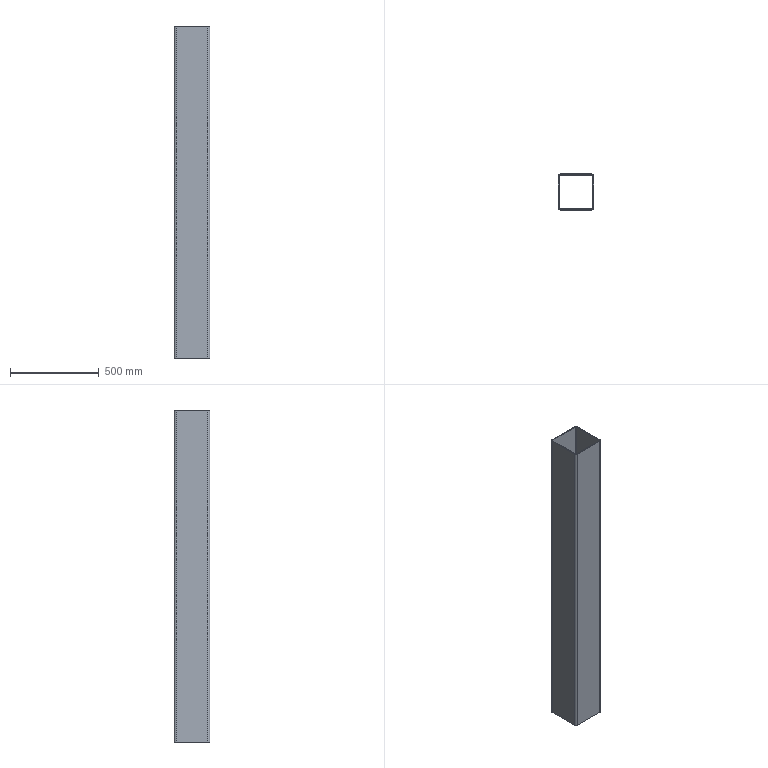Component | SolidWorks | 200 x 200 x 5-1 | 1 solid | 18 faces | box 200 x 200 x 1874 mm | volume 7187951 mm3 | plane 10 | cylinder 8 | commonest cylinder face diameters 20 x4 10 x4 | material Plain Carbon Steel
build123d program:
from build123d import *

# Parameters (mm, degrees)
BOSS_EXTRUDE1_DEPTH = 1874


with BuildPart() as part:
    # Sketch1 → Boss-Extrude1 (new body)
    with BuildSketch(Plane.XY):
        with BuildLine():
            Line((-90, -100), (90, -100))
            ThreePointArc((90, -100), (97.071, -97.071), (100, -90))
            Line((100, -90), (100, 90))
            ThreePointArc((100, 90), (97.071, 97.071), (90, 100))
            Line((90, 100), (-90, 100))
            ThreePointArc((-90, 100), (-97.071, 97.071), (-100, 90))
            Line((-100, 90), (-100, -90))
            ThreePointArc((-100, -90), (-97.071, -97.071), (-90, -100))
        make_face()
        with BuildLine():
            Line((-90, -95), (90, -95))
            ThreePointArc((90, -95), (93.536, -93.536), (95, -90))
            Line((95, -90), (95, 90))
            ThreePointArc((95, 90), (93.536, 93.536), (90, 95))
            Line((90, 95), (-90, 95))
            ThreePointArc((-90, 95), (-93.536, 93.536), (-95, 90))
            Line((-95, 90), (-95, -90))
            ThreePointArc((-95, -90), (-93.536, -93.536), (-90, -95))
        make_face(mode=Mode.SUBTRACT)
    extrude(amount=BOSS_EXTRUDE1_DEPTH)


solid = part.part

# Placed as in the assembly
solid = solid.moved(Location((585.937, 2371.697, 1863.287), (0, 0, 0)))
STEP:
#1=CARTESIAN_POINT('',(19.131,89.831,147.137));
#2=VERTEX_POINT('',#1);
#3=CARTESIAN_POINT('',(19.525,89.437,147.137));
#4=VERTEX_POINT('',#3);
#5=CARTESIAN_POINT('',(19.525,89.831,147.137));
#6=DIRECTION('',(0.,0.,1.));
#7=DIRECTION('',(1.,0.,0.));
#8=AXIS2_PLACEMENT_3D('',#5,#6,#7);
#9=CIRCLE('',#8,0.3937);
#10=EDGE_CURVE('',#2,#4,#9,.T.);
#11=ORIENTED_EDGE('',*,*,#10,.T.);
#12=CARTESIAN_POINT('',(26.612,89.437,147.137));
#13=VERTEX_POINT('',#12);
#14=CARTESIAN_POINT('',(19.525,89.437,147.137));
#15=DIRECTION('',(1.,0.,0.));
#16=VECTOR('',#15,39.37);
#17=LINE('',#14,#16);
#18=EDGE_CURVE('',#4,#13,#17,.T.);
#19=ORIENTED_EDGE('',*,*,#18,.T.);
#20=CARTESIAN_POINT('',(27.005,89.831,147.137));
#21=VERTEX_POINT('',#20);
#22=CARTESIAN_POINT('',(26.612,89.831,147.137));
#23=DIRECTION('',(0.,0.,1.));
#24=DIRECTION('',(1.,0.,0.));
#25=AXIS2_PLACEMENT_3D('',#22,#23,#24);
#26=CIRCLE('',#25,0.3937);
#27=EDGE_CURVE('',#13,#21,#26,.T.);
#28=ORIENTED_EDGE('',*,*,#27,.T.);
#29=CARTESIAN_POINT('',(27.005,96.917,147.137));
#30=VERTEX_POINT('',#29);
#31=CARTESIAN_POINT('',(27.005,96.917,147.137));
#32=DIRECTION('',(0.,-1.,0.));
#33=VECTOR('',#32,39.37);
#34=LINE('',#31,#33);
#35=EDGE_CURVE('',#30,#21,#34,.T.);
#36=ORIENTED_EDGE('',*,*,#35,.F.);
#37=CARTESIAN_POINT('',(26.612,97.311,147.137));
#38=VERTEX_POINT('',#37);
#39=CARTESIAN_POINT('',(26.612,96.917,147.137));
#40=DIRECTION('',(0.,0.,1.));
#41=DIRECTION('',(1.,0.,0.));
#42=AXIS2_PLACEMENT_3D('',#39,#40,#41);
#43=CIRCLE('',#42,0.3937);
#44=EDGE_CURVE('',#30,#38,#43,.T.);
#45=ORIENTED_EDGE('',*,*,#44,.T.);
#46=CARTESIAN_POINT('',(19.525,97.311,147.137));
#47=VERTEX_POINT('',#46);
#48=CARTESIAN_POINT('',(26.612,97.311,147.137));
#49=DIRECTION('',(-1.,0.,0.));
#50=VECTOR('',#49,39.37);
#51=LINE('',#48,#50);
#52=EDGE_CURVE('',#38,#47,#51,.T.);
#53=ORIENTED_EDGE('',*,*,#52,.T.);
#54=CARTESIAN_POINT('',(19.131,96.917,147.137));
#55=VERTEX_POINT('',#54);
#56=CARTESIAN_POINT('',(19.525,96.917,147.137));
#57=DIRECTION('',(0.,0.,1.));
#58=DIRECTION('',(1.,0.,0.));
#59=AXIS2_PLACEMENT_3D('',#56,#57,#58);
#60=CIRCLE('',#59,0.3937);
#61=EDGE_CURVE('',#47,#55,#60,.T.);
#62=ORIENTED_EDGE('',*,*,#61,.T.);
#63=CARTESIAN_POINT('',(19.131,89.831,147.137));
#64=DIRECTION('',(0.,1.,0.));
#65=VECTOR('',#64,39.37);
#66=LINE('',#63,#65);
#67=EDGE_CURVE('',#2,#55,#66,.T.);
#68=ORIENTED_EDGE('',*,*,#67,.F.);
#69=EDGE_LOOP('',(#11,#19,#28,#36,#45,#53,#62,#68));
#70=FACE_OUTER_BOUND('',#69,.T.);
#71=CARTESIAN_POINT('',(19.525,89.634,147.137));
#72=VERTEX_POINT('',#71);
#73=CARTESIAN_POINT('',(26.612,89.634,147.137));
#74=VERTEX_POINT('',#73);
#75=CARTESIAN_POINT('',(19.525,89.634,147.137));
#76=DIRECTION('',(1.,0.,0.));
#77=VECTOR('',#76,39.37);
#78=LINE('',#75,#77);
#79=EDGE_CURVE('',#72,#74,#78,.T.);
#80=ORIENTED_EDGE('',*,*,#79,.F.);
#81=CARTESIAN_POINT('',(19.328,89.831,147.137));
#82=VERTEX_POINT('',#81);
#83=CARTESIAN_POINT('',(19.525,89.831,147.137));
#84=DIRECTION('',(0.,0.,1.));
#85=DIRECTION('',(1.,0.,0.));
#86=AXIS2_PLACEMENT_3D('',#83,#84,#85);
#87=CIRCLE('',#86,0.1969);
#88=EDGE_CURVE('',#82,#72,#87,.T.);
#89=ORIENTED_EDGE('',*,*,#88,.F.);
#90=CARTESIAN_POINT('',(19.328,96.917,147.137));
#91=VERTEX_POINT('',#90);
#92=CARTESIAN_POINT('',(19.328,89.831,147.137));
#93=DIRECTION('',(0.,1.,0.));
#94=VECTOR('',#93,39.37);
#95=LINE('',#92,#94);
#96=EDGE_CURVE('',#82,#91,#95,.T.);
#97=ORIENTED_EDGE('',*,*,#96,.T.);
#98=CARTESIAN_POINT('',(19.525,97.114,147.137));
#99=VERTEX_POINT('',#98);
#100=CARTESIAN_POINT('',(19.525,96.917,147.137));
#101=DIRECTION('',(0.,0.,1.));
#102=DIRECTION('',(1.,0.,0.));
#103=AXIS2_PLACEMENT_3D('',#100,#101,#102);
#104=CIRCLE('',#103,0.1969);
#105=EDGE_CURVE('',#99,#91,#104,.T.);
#106=ORIENTED_EDGE('',*,*,#105,.F.);
#107=CARTESIAN_POINT('',(26.612,97.114,147.137));
#108=VERTEX_POINT('',#107);
#109=CARTESIAN_POINT('',(26.612,97.114,147.137));
#110=DIRECTION('',(-1.,0.,0.));
#111=VECTOR('',#110,39.37);
#112=LINE('',#109,#111);
#113=EDGE_CURVE('',#108,#99,#112,.T.);
#114=ORIENTED_EDGE('',*,*,#113,.F.);
#115=CARTESIAN_POINT('',(26.809,96.917,147.137));
#116=VERTEX_POINT('',#115);
#117=CARTESIAN_POINT('',(26.612,96.917,147.137));
#118=DIRECTION('',(0.,0.,1.));
#119=DIRECTION('',(1.,0.,0.));
#120=AXIS2_PLACEMENT_3D('',#117,#118,#119);
#121=CIRCLE('',#120,0.1969);
#122=EDGE_CURVE('',#116,#108,#121,.T.);
#123=ORIENTED_EDGE('',*,*,#122,.F.);
#124=CARTESIAN_POINT('',(26.809,89.831,147.137));
#125=VERTEX_POINT('',#124);
#126=CARTESIAN_POINT('',(26.809,96.917,147.137));
#127=DIRECTION('',(0.,-1.,0.));
#128=VECTOR('',#127,39.37);
#129=LINE('',#126,#128);
#130=EDGE_CURVE('',#116,#125,#129,.T.);
#131=ORIENTED_EDGE('',*,*,#130,.T.);
#132=CARTESIAN_POINT('',(26.612,89.831,147.137));
#133=DIRECTION('',(0.,0.,1.));
#134=DIRECTION('',(1.,0.,0.));
#135=AXIS2_PLACEMENT_3D('',#132,#133,#134);
#136=CIRCLE('',#135,0.1969);
#137=EDGE_CURVE('',#74,#125,#136,.T.);
#138=ORIENTED_EDGE('',*,*,#137,.F.);
#139=EDGE_LOOP('',(#80,#89,#97,#106,#114,#123,#131,#138));
#140=FACE_BOUND('',#139,.T.);
#141=CARTESIAN_POINT('',(19.525,89.831,147.137));
#142=DIRECTION('',(0.,0.,1.));
#143=DIRECTION('',(1.,0.,0.));
#144=AXIS2_PLACEMENT_3D('',#141,#142,#143);
#145=PLANE('',#144);
#146=ADVANCED_FACE('',(#70,#140),#145,.T.);
#147=CARTESIAN_POINT('',(19.131,89.831,73.358));
#148=VERTEX_POINT('',#147);
#149=CARTESIAN_POINT('',(19.525,89.437,73.358));
#150=VERTEX_POINT('',#149);
#151=CARTESIAN_POINT('',(19.525,89.831,73.358));
#152=DIRECTION('',(0.,0.,1.));
#153=DIRECTION('',(1.,0.,0.));
#154=AXIS2_PLACEMENT_3D('',#151,#152,#153);
#155=CIRCLE('',#154,0.3937);
#156=EDGE_CURVE('',#148,#150,#155,.T.);
#157=ORIENTED_EDGE('',*,*,#156,.F.);
#158=CARTESIAN_POINT('',(19.131,96.917,73.358));
#159=VERTEX_POINT('',#158);
#160=CARTESIAN_POINT('',(19.131,89.831,73.358));
#161=DIRECTION('',(0.,1.,0.));
#162=VECTOR('',#161,39.37);
#163=LINE('',#160,#162);
#164=EDGE_CURVE('',#148,#159,#163,.T.);
#165=ORIENTED_EDGE('',*,*,#164,.T.);
#166=CARTESIAN_POINT('',(19.525,97.311,73.358));
#167=VERTEX_POINT('',#166);
#168=CARTESIAN_POINT('',(19.525,96.917,73.358));
#169=DIRECTION('',(0.,0.,1.));
#170=DIRECTION('',(1.,0.,0.));
#171=AXIS2_PLACEMENT_3D('',#168,#169,#170);
#172=CIRCLE('',#171,0.3937);
#173=EDGE_CURVE('',#167,#159,#172,.T.);
#174=ORIENTED_EDGE('',*,*,#173,.F.);
#175=CARTESIAN_POINT('',(26.612,97.311,73.358));
#176=VERTEX_POINT('',#175);
#177=CARTESIAN_POINT('',(26.612,97.311,73.358));
#178=DIRECTION('',(-1.,0.,0.));
#179=VECTOR('',#178,39.37);
#180=LINE('',#177,#179);
#181=EDGE_CURVE('',#176,#167,#180,.T.);
#182=ORIENTED_EDGE('',*,*,#181,.F.);
#183=CARTESIAN_POINT('',(27.005,96.917,73.358));
#184=VERTEX_POINT('',#183);
#185=CARTESIAN_POINT('',(26.612,96.917,73.358));
#186=DIRECTION('',(0.,0.,1.));
#187=DIRECTION('',(1.,0.,0.));
#188=AXIS2_PLACEMENT_3D('',#185,#186,#187);
#189=CIRCLE('',#188,0.3937);
#190=EDGE_CURVE('',#184,#176,#189,.T.);
#191=ORIENTED_EDGE('',*,*,#190,.F.);
#192=CARTESIAN_POINT('',(27.005,89.831,73.358));
#193=VERTEX_POINT('',#192);
#194=CARTESIAN_POINT('',(27.005,96.917,73.358));
#195=DIRECTION('',(0.,-1.,0.));
#196=VECTOR('',#195,39.37);
#197=LINE('',#194,#196);
#198=EDGE_CURVE('',#184,#193,#197,.T.);
#199=ORIENTED_EDGE('',*,*,#198,.T.);
#200=CARTESIAN_POINT('',(26.612,89.437,73.358));
#201=VERTEX_POINT('',#200);
#202=CARTESIAN_POINT('',(26.612,89.831,73.358));
#203=DIRECTION('',(0.,0.,1.));
#204=DIRECTION('',(1.,0.,0.));
#205=AXIS2_PLACEMENT_3D('',#202,#203,#204);
#206=CIRCLE('',#205,0.3937);
#207=EDGE_CURVE('',#201,#193,#206,.T.);
#208=ORIENTED_EDGE('',*,*,#207,.F.);
#209=CARTESIAN_POINT('',(19.525,89.437,73.358));
#210=DIRECTION('',(1.,0.,0.));
#211=VECTOR('',#210,39.37);
#212=LINE('',#209,#211);
#213=EDGE_CURVE('',#150,#201,#212,.T.);
#214=ORIENTED_EDGE('',*,*,#213,.F.);
#215=EDGE_LOOP('',(#157,#165,#174,#182,#191,#199,#208,#214));
#216=FACE_OUTER_BOUND('',#215,.T.);
#217=CARTESIAN_POINT('',(19.328,89.831,73.358));
#218=VERTEX_POINT('',#217);
#219=CARTESIAN_POINT('',(19.525,89.634,73.358));
#220=VERTEX_POINT('',#219);
#221=CARTESIAN_POINT('',(19.525,89.831,73.358));
#222=DIRECTION('',(0.,0.,1.));
#223=DIRECTION('',(1.,0.,0.));
#224=AXIS2_PLACEMENT_3D('',#221,#222,#223);
#225=CIRCLE('',#224,0.1969);
#226=EDGE_CURVE('',#218,#220,#225,.T.);
#227=ORIENTED_EDGE('',*,*,#226,.T.);
#228=CARTESIAN_POINT('',(26.612,89.634,73.358));
#229=VERTEX_POINT('',#228);
#230=CARTESIAN_POINT('',(19.525,89.634,73.358));
#231=DIRECTION('',(1.,0.,0.));
#232=VECTOR('',#231,39.37);
#233=LINE('',#230,#232);
#234=EDGE_CURVE('',#220,#229,#233,.T.);
#235=ORIENTED_EDGE('',*,*,#234,.T.);
#236=CARTESIAN_POINT('',(26.809,89.831,73.358));
#237=VERTEX_POINT('',#236);
#238=CARTESIAN_POINT('',(26.612,89.831,73.358));
#239=DIRECTION('',(0.,0.,1.));
#240=DIRECTION('',(1.,0.,0.));
#241=AXIS2_PLACEMENT_3D('',#238,#239,#240);
#242=CIRCLE('',#241,0.1969);
#243=EDGE_CURVE('',#229,#237,#242,.T.);
#244=ORIENTED_EDGE('',*,*,#243,.T.);
#245=CARTESIAN_POINT('',(26.809,96.917,73.358));
#246=VERTEX_POINT('',#245);
#247=CARTESIAN_POINT('',(26.809,96.917,73.358));
#248=DIRECTION('',(0.,-1.,0.));
#249=VECTOR('',#248,39.37);
#250=LINE('',#247,#249);
#251=EDGE_CURVE('',#246,#237,#250,.T.);
#252=ORIENTED_EDGE('',*,*,#251,.F.);
#253=CARTESIAN_POINT('',(26.612,97.114,73.358));
#254=VERTEX_POINT('',#253);
#255=CARTESIAN_POINT('',(26.612,96.917,73.358));
#256=DIRECTION('',(0.,0.,1.));
#257=DIRECTION('',(1.,0.,0.));
#258=AXIS2_PLACEMENT_3D('',#255,#256,#257);
#259=CIRCLE('',#258,0.1969);
#260=EDGE_CURVE('',#246,#254,#259,.T.);
#261=ORIENTED_EDGE('',*,*,#260,.T.);
#262=CARTESIAN_POINT('',(19.525,97.114,73.358));
#263=VERTEX_POINT('',#262);
#264=CARTESIAN_POINT('',(26.612,97.114,73.358));
#265=DIRECTION('',(-1.,0.,0.));
#266=VECTOR('',#265,39.37);
#267=LINE('',#264,#266);
#268=EDGE_CURVE('',#254,#263,#267,.T.);
#269=ORIENTED_EDGE('',*,*,#268,.T.);
#270=CARTESIAN_POINT('',(19.328,96.917,73.358));
#271=VERTEX_POINT('',#270);
#272=CARTESIAN_POINT('',(19.525,96.917,73.358));
#273=DIRECTION('',(0.,0.,1.));
#274=DIRECTION('',(1.,0.,0.));
#275=AXIS2_PLACEMENT_3D('',#272,#273,#274);
#276=CIRCLE('',#275,0.1969);
#277=EDGE_CURVE('',#263,#271,#276,.T.);
#278=ORIENTED_EDGE('',*,*,#277,.T.);
#279=CARTESIAN_POINT('',(19.328,89.831,73.358));
#280=DIRECTION('',(0.,1.,0.));
#281=VECTOR('',#280,39.37);
#282=LINE('',#279,#281);
#283=EDGE_CURVE('',#218,#271,#282,.T.);
#284=ORIENTED_EDGE('',*,*,#283,.F.);
#285=EDGE_LOOP('',(#227,#235,#244,#252,#261,#269,#278,#284));
#286=FACE_BOUND('',#285,.T.);
#287=CARTESIAN_POINT('',(19.525,89.831,73.358));
#288=DIRECTION('',(0.,0.,1.));
#289=DIRECTION('',(1.,0.,0.));
#290=AXIS2_PLACEMENT_3D('',#287,#288,#289);
#291=PLANE('',#290);
#292=ADVANCED_FACE('',(#216,#286),#291,.F.);
#293=ORIENTED_EDGE('',*,*,#156,.T.);
#294=CARTESIAN_POINT('',(19.525,89.437,147.137));
#295=DIRECTION('',(0.,0.,-1.));
#296=VECTOR('',#295,39.37);
#297=LINE('',#294,#296);
#298=EDGE_CURVE('',#4,#150,#297,.T.);
#299=ORIENTED_EDGE('',*,*,#298,.F.);
#300=ORIENTED_EDGE('',*,*,#10,.F.);
#301=CARTESIAN_POINT('',(19.131,89.831,147.137));
#302=DIRECTION('',(0.,0.,-1.));
#303=VECTOR('',#302,39.37);
#304=LINE('',#301,#303);
#305=EDGE_CURVE('',#2,#148,#304,.T.);
#306=ORIENTED_EDGE('',*,*,#305,.T.);
#307=EDGE_LOOP('',(#293,#299,#300,#306));
#308=FACE_OUTER_BOUND('',#307,.T.);
#309=CARTESIAN_POINT('',(19.525,89.831,147.137));
#310=DIRECTION('',(0.,0.,-1.));
#311=DIRECTION('',(-1.,0.,0.));
#312=AXIS2_PLACEMENT_3D('',#309,#310,#311);
#313=CYLINDRICAL_SURFACE('',#312,0.3937);
#314=ADVANCED_FACE('',(#308),#313,.T.);
#315=ORIENTED_EDGE('',*,*,#213,.T.);
#316=CARTESIAN_POINT('',(26.612,89.437,147.137));
#317=DIRECTION('',(0.,0.,-1.));
#318=VECTOR('',#317,39.37);
#319=LINE('',#316,#318);
#320=EDGE_CURVE('',#13,#201,#319,.T.);
#321=ORIENTED_EDGE('',*,*,#320,.F.);
#322=ORIENTED_EDGE('',*,*,#18,.F.);
#323=ORIENTED_EDGE('',*,*,#298,.T.);
#324=EDGE_LOOP('',(#315,#321,#322,#323));
#325=FACE_OUTER_BOUND('',#324,.T.);
#326=CARTESIAN_POINT('',(19.525,89.437,147.137));
#327=DIRECTION('',(0.,1.,0.));
#328=DIRECTION('',(0.,0.,1.));
#329=AXIS2_PLACEMENT_3D('',#326,#327,#328);
#330=PLANE('',#329);
#331=ADVANCED_FACE('',(#325),#330,.F.);
#332=ORIENTED_EDGE('',*,*,#207,.T.);
#333=CARTESIAN_POINT('',(27.005,89.831,147.137));
#334=DIRECTION('',(0.,0.,-1.));
#335=VECTOR('',#334,39.37);
#336=LINE('',#333,#335);
#337=EDGE_CURVE('',#21,#193,#336,.T.);
#338=ORIENTED_EDGE('',*,*,#337,.F.);
#339=ORIENTED_EDGE('',*,*,#27,.F.);
#340=ORIENTED_EDGE('',*,*,#320,.T.);
#341=EDGE_LOOP('',(#332,#338,#339,#340));
#342=FACE_OUTER_BOUND('',#341,.T.);
#343=CARTESIAN_POINT('',(26.612,89.831,147.137));
#344=DIRECTION('',(0.,0.,-1.));
#345=DIRECTION('',(-1.,0.,0.));
#346=AXIS2_PLACEMENT_3D('',#343,#344,#345);
#347=CYLINDRICAL_SURFACE('',#346,0.3937);
#348=ADVANCED_FACE('',(#342),#347,.T.);
#349=ORIENTED_EDGE('',*,*,#198,.F.);
#350=CARTESIAN_POINT('',(27.005,96.917,147.137));
#351=DIRECTION('',(0.,0.,-1.));
#352=VECTOR('',#351,39.37);
#353=LINE('',#350,#352);
#354=EDGE_CURVE('',#30,#184,#353,.T.);
#355=ORIENTED_EDGE('',*,*,#354,.F.);
#356=ORIENTED_EDGE('',*,*,#35,.T.);
#357=ORIENTED_EDGE('',*,*,#337,.T.);
#358=EDGE_LOOP('',(#349,#355,#356,#357));
#359=FACE_OUTER_BOUND('',#358,.T.);
#360=CARTESIAN_POINT('',(27.005,96.917,147.137));
#361=DIRECTION('',(1.,0.,0.));
#362=DIRECTION('',(0.,0.,-1.));
#363=AXIS2_PLACEMENT_3D('',#360,#361,#362);
#364=PLANE('',#363);
#365=ADVANCED_FACE('',(#359),#364,.T.);
#366=ORIENTED_EDGE('',*,*,#190,.T.);
#367=CARTESIAN_POINT('',(26.612,97.311,147.137));
#368=DIRECTION('',(0.,0.,-1.));
#369=VECTOR('',#368,39.37);
#370=LINE('',#367,#369);
#371=EDGE_CURVE('',#38,#176,#370,.T.);
#372=ORIENTED_EDGE('',*,*,#371,.F.);
#373=ORIENTED_EDGE('',*,*,#44,.F.);
#374=ORIENTED_EDGE('',*,*,#354,.T.);
#375=EDGE_LOOP('',(#366,#372,#373,#374));
#376=FACE_OUTER_BOUND('',#375,.T.);
#377=CARTESIAN_POINT('',(26.612,96.917,147.137));
#378=DIRECTION('',(0.,0.,-1.));
#379=DIRECTION('',(-1.,0.,0.));
#380=AXIS2_PLACEMENT_3D('',#377,#378,#379);
#381=CYLINDRICAL_SURFACE('',#380,0.3937);
#382=ADVANCED_FACE('',(#376),#381,.T.);
#383=ORIENTED_EDGE('',*,*,#181,.T.);
#384=CARTESIAN_POINT('',(19.525,97.311,147.137));
#385=DIRECTION('',(0.,0.,-1.));
#386=VECTOR('',#385,39.37);
#387=LINE('',#384,#386);
#388=EDGE_CURVE('',#47,#167,#387,.T.);
#389=ORIENTED_EDGE('',*,*,#388,.F.);
#390=ORIENTED_EDGE('',*,*,#52,.F.);
#391=ORIENTED_EDGE('',*,*,#371,.T.);
#392=EDGE_LOOP('',(#383,#389,#390,#391));
#393=FACE_OUTER_BOUND('',#392,.T.);
#394=CARTESIAN_POINT('',(26.612,97.311,147.137));
#395=DIRECTION('',(0.,-1.,0.));
#396=DIRECTION('',(0.,0.,-1.));
#397=AXIS2_PLACEMENT_3D('',#394,#395,#396);
#398=PLANE('',#397);
#399=ADVANCED_FACE('',(#393),#398,.F.);
#400=ORIENTED_EDGE('',*,*,#173,.T.);
#401=CARTESIAN_POINT('',(19.131,96.917,147.137));
#402=DIRECTION('',(0.,0.,-1.));
#403=VECTOR('',#402,39.37);
#404=LINE('',#401,#403);
#405=EDGE_CURVE('',#55,#159,#404,.T.);
#406=ORIENTED_EDGE('',*,*,#405,.F.);
#407=ORIENTED_EDGE('',*,*,#61,.F.);
#408=ORIENTED_EDGE('',*,*,#388,.T.);
#409=EDGE_LOOP('',(#400,#406,#407,#408));
#410=FACE_OUTER_BOUND('',#409,.T.);
#411=CARTESIAN_POINT('',(19.525,96.917,147.137));
#412=DIRECTION('',(0.,0.,-1.));
#413=DIRECTION('',(-1.,0.,0.));
#414=AXIS2_PLACEMENT_3D('',#411,#412,#413);
#415=CYLINDRICAL_SURFACE('',#414,0.3937);
#416=ADVANCED_FACE('',(#410),#415,.T.);
#417=ORIENTED_EDGE('',*,*,#164,.F.);
#418=ORIENTED_EDGE('',*,*,#305,.F.);
#419=ORIENTED_EDGE('',*,*,#67,.T.);
#420=ORIENTED_EDGE('',*,*,#405,.T.);
#421=EDGE_LOOP('',(#417,#418,#419,#420));
#422=FACE_OUTER_BOUND('',#421,.T.);
#423=CARTESIAN_POINT('',(19.131,89.831,147.137));
#424=DIRECTION('',(-1.,0.,0.));
#425=DIRECTION('',(0.,0.,1.));
#426=AXIS2_PLACEMENT_3D('',#423,#424,#425);
#427=PLANE('',#426);
#428=ADVANCED_FACE('',(#422),#427,.T.);
#429=ORIENTED_EDGE('',*,*,#226,.F.);
#430=CARTESIAN_POINT('',(19.328,89.831,147.137));
#431=DIRECTION('',(0.,0.,-1.));
#432=VECTOR('',#431,39.37);
#433=LINE('',#430,#432);
#434=EDGE_CURVE('',#82,#218,#433,.T.);
#435=ORIENTED_EDGE('',*,*,#434,.F.);
#436=ORIENTED_EDGE('',*,*,#88,.T.);
#437=CARTESIAN_POINT('',(19.525,89.634,147.137));
#438=DIRECTION('',(0.,0.,-1.));
#439=VECTOR('',#438,39.37);
#440=LINE('',#437,#439);
#441=EDGE_CURVE('',#72,#220,#440,.T.);
#442=ORIENTED_EDGE('',*,*,#441,.T.);
#443=EDGE_LOOP('',(#429,#435,#436,#442));
#444=FACE_OUTER_BOUND('',#443,.T.);
#445=CARTESIAN_POINT('',(19.525,89.831,147.137));
#446=DIRECTION('',(0.,0.,-1.));
#447=DIRECTION('',(-1.,0.,0.));
#448=AXIS2_PLACEMENT_3D('',#445,#446,#447);
#449=CYLINDRICAL_SURFACE('',#448,0.1969);
#450=ADVANCED_FACE('',(#444),#449,.F.);
#451=ORIENTED_EDGE('',*,*,#234,.F.);
#452=ORIENTED_EDGE('',*,*,#441,.F.);
#453=ORIENTED_EDGE('',*,*,#79,.T.);
#454=CARTESIAN_POINT('',(26.612,89.634,147.137));
#455=DIRECTION('',(0.,0.,-1.));
#456=VECTOR('',#455,39.37);
#457=LINE('',#454,#456);
#458=EDGE_CURVE('',#74,#229,#457,.T.);
#459=ORIENTED_EDGE('',*,*,#458,.T.);
#460=EDGE_LOOP('',(#451,#452,#453,#459));
#461=FACE_OUTER_BOUND('',#460,.T.);
#462=CARTESIAN_POINT('',(19.525,89.634,147.137));
#463=DIRECTION('',(0.,1.,0.));
#464=DIRECTION('',(0.,0.,1.));
#465=AXIS2_PLACEMENT_3D('',#462,#463,#464);
#466=PLANE('',#465);
#467=ADVANCED_FACE('',(#461),#466,.T.);
#468=ORIENTED_EDGE('',*,*,#243,.F.);
#469=ORIENTED_EDGE('',*,*,#458,.F.);
#470=ORIENTED_EDGE('',*,*,#137,.T.);
#471=CARTESIAN_POINT('',(26.809,89.831,147.137));
#472=DIRECTION('',(0.,0.,-1.));
#473=VECTOR('',#472,39.37);
#474=LINE('',#471,#473);
#475=EDGE_CURVE('',#125,#237,#474,.T.);
#476=ORIENTED_EDGE('',*,*,#475,.T.);
#477=EDGE_LOOP('',(#468,#469,#470,#476));
#478=FACE_OUTER_BOUND('',#477,.T.);
#479=CARTESIAN_POINT('',(26.612,89.831,147.137));
#480=DIRECTION('',(0.,0.,-1.));
#481=DIRECTION('',(-1.,0.,0.));
#482=AXIS2_PLACEMENT_3D('',#479,#480,#481);
#483=CYLINDRICAL_SURFACE('',#482,0.1969);
#484=ADVANCED_FACE('',(#478),#483,.F.);
#485=ORIENTED_EDGE('',*,*,#251,.T.);
#486=ORIENTED_EDGE('',*,*,#475,.F.);
#487=ORIENTED_EDGE('',*,*,#130,.F.);
#488=CARTESIAN_POINT('',(26.809,96.917,147.137));
#489=DIRECTION('',(0.,0.,-1.));
#490=VECTOR('',#489,39.37);
#491=LINE('',#488,#490);
#492=EDGE_CURVE('',#116,#246,#491,.T.);
#493=ORIENTED_EDGE('',*,*,#492,.T.);
#494=EDGE_LOOP('',(#485,#486,#487,#493));
#495=FACE_OUTER_BOUND('',#494,.T.);
#496=CARTESIAN_POINT('',(26.809,96.917,147.137));
#497=DIRECTION('',(1.,0.,0.));
#498=DIRECTION('',(0.,0.,-1.));
#499=AXIS2_PLACEMENT_3D('',#496,#497,#498);
#500=PLANE('',#499);
#501=ADVANCED_FACE('',(#495),#500,.F.);
#502=ORIENTED_EDGE('',*,*,#260,.F.);
#503=ORIENTED_EDGE('',*,*,#492,.F.);
#504=ORIENTED_EDGE('',*,*,#122,.T.);
#505=CARTESIAN_POINT('',(26.612,97.114,147.137));
#506=DIRECTION('',(0.,0.,-1.));
#507=VECTOR('',#506,39.37);
#508=LINE('',#505,#507);
#509=EDGE_CURVE('',#108,#254,#508,.T.);
#510=ORIENTED_EDGE('',*,*,#509,.T.);
#511=EDGE_LOOP('',(#502,#503,#504,#510));
#512=FACE_OUTER_BOUND('',#511,.T.);
#513=CARTESIAN_POINT('',(26.612,96.917,147.137));
#514=DIRECTION('',(0.,0.,-1.));
#515=DIRECTION('',(-1.,0.,0.));
#516=AXIS2_PLACEMENT_3D('',#513,#514,#515);
#517=CYLINDRICAL_SURFACE('',#516,0.1969);
#518=ADVANCED_FACE('',(#512),#517,.F.);
#519=ORIENTED_EDGE('',*,*,#268,.F.);
#520=ORIENTED_EDGE('',*,*,#509,.F.);
#521=ORIENTED_EDGE('',*,*,#113,.T.);
#522=CARTESIAN_POINT('',(19.525,97.114,147.137));
#523=DIRECTION('',(0.,0.,-1.));
#524=VECTOR('',#523,39.37);
#525=LINE('',#522,#524);
#526=EDGE_CURVE('',#99,#263,#525,.T.);
#527=ORIENTED_EDGE('',*,*,#526,.T.);
#528=EDGE_LOOP('',(#519,#520,#521,#527));
#529=FACE_OUTER_BOUND('',#528,.T.);
#530=CARTESIAN_POINT('',(26.612,97.114,147.137));
#531=DIRECTION('',(0.,-1.,0.));
#532=DIRECTION('',(0.,0.,-1.));
#533=AXIS2_PLACEMENT_3D('',#530,#531,#532);
#534=PLANE('',#533);
#535=ADVANCED_FACE('',(#529),#534,.T.);
#536=ORIENTED_EDGE('',*,*,#277,.F.);
#537=ORIENTED_EDGE('',*,*,#526,.F.);
#538=ORIENTED_EDGE('',*,*,#105,.T.);
#539=CARTESIAN_POINT('',(19.328,96.917,147.137));
#540=DIRECTION('',(0.,0.,-1.));
#541=VECTOR('',#540,39.37);
#542=LINE('',#539,#541);
#543=EDGE_CURVE('',#91,#271,#542,.T.);
#544=ORIENTED_EDGE('',*,*,#543,.T.);
#545=EDGE_LOOP('',(#536,#537,#538,#544));
#546=FACE_OUTER_BOUND('',#545,.T.);
#547=CARTESIAN_POINT('',(19.525,96.917,147.137));
#548=DIRECTION('',(0.,0.,-1.));
#549=DIRECTION('',(-1.,0.,0.));
#550=AXIS2_PLACEMENT_3D('',#547,#548,#549);
#551=CYLINDRICAL_SURFACE('',#550,0.1969);
#552=ADVANCED_FACE('',(#546),#551,.F.);
#553=ORIENTED_EDGE('',*,*,#283,.T.);
#554=ORIENTED_EDGE('',*,*,#543,.F.);
#555=ORIENTED_EDGE('',*,*,#96,.F.);
#556=ORIENTED_EDGE('',*,*,#434,.T.);
#557=EDGE_LOOP('',(#553,#554,#555,#556));
#558=FACE_OUTER_BOUND('',#557,.T.);
#559=CARTESIAN_POINT('',(19.328,89.831,147.137));
#560=DIRECTION('',(-1.,0.,0.));
#561=DIRECTION('',(0.,0.,1.));
#562=AXIS2_PLACEMENT_3D('',#559,#560,#561);
#563=PLANE('',#562);
#564=ADVANCED_FACE('',(#558),#563,.F.);
#565=CLOSED_SHELL('',(#146,#292,#314,#331,#348,#365,#382,#399,#416,#428,#450,#467,#484,#501,#518,#535,#552,#564));
#566=MANIFOLD_SOLID_BREP('',#565);
#567=CARTESIAN_POINT('',(0.,0.,0.));
#568=DIRECTION('',(0.,0.,1.));
#569=DIRECTION('',(1.,0.,0.));
#570=AXIS2_PLACEMENT_3D('',#567,#568,#569);
#571=(LENGTH_UNIT()NAMED_UNIT(*)SI_UNIT($,.METRE.));
#572=LENGTH_MEASURE_WITH_UNIT(LENGTH_MEASURE(0.0254),#571);
#573=DIMENSIONAL_EXPONENTS(1.,0.,0.,0.,0.,0.,0.);
#574=(CONVERSION_BASED_UNIT('',#572)LENGTH_UNIT()NAMED_UNIT(#573));
#575=UNCERTAINTY_MEASURE_WITH_UNIT(LENGTH_MEASURE(0.00001),#574,'','');
#576=(NAMED_UNIT(*)PLANE_ANGLE_UNIT()SI_UNIT($,.RADIAN.));
#577=(NAMED_UNIT(*)SI_UNIT($,.STERADIAN.)SOLID_ANGLE_UNIT());
#578=(GEOMETRIC_REPRESENTATION_CONTEXT(3)GLOBAL_UNCERTAINTY_ASSIGNED_CONTEXT((#575))GLOBAL_UNIT_ASSIGNED_CONTEXT((#574,#576,#577))REPRESENTATION_CONTEXT('',''));
#579=ADVANCED_BREP_SHAPE_REPRESENTATION('',(#566,#570),#578);
#580=COLOUR_RGB('',0.7922,0.8196,0.9333);
#581=FILL_AREA_STYLE_COLOUR('',#580);
#582=FILL_AREA_STYLE('',(#581));
#583=SURFACE_STYLE_FILL_AREA(#582);
#584=SURFACE_SIDE_STYLE('',(#583));
#585=SURFACE_STYLE_USAGE(.BOTH.,#584);
#586=PRESENTATION_STYLE_ASSIGNMENT((#585));
#587=STYLED_ITEM('',(#586),#566);
#588=PRESENTATION_LAYER_ASSIGNMENT('','',(#587));
#589=(LENGTH_UNIT()NAMED_UNIT(*)SI_UNIT($,.METRE.));
#590=LENGTH_MEASURE_WITH_UNIT(LENGTH_MEASURE(0.0254),#589);
#591=DIMENSIONAL_EXPONENTS(1.,0.,0.,0.,0.,0.,0.);
#592=(CONVERSION_BASED_UNIT('',#590)LENGTH_UNIT()NAMED_UNIT(#591));
#593=UNCERTAINTY_MEASURE_WITH_UNIT(LENGTH_MEASURE(0.00001),#592,'','');
#594=(NAMED_UNIT(*)PLANE_ANGLE_UNIT()SI_UNIT($,.RADIAN.));
#595=(NAMED_UNIT(*)SI_UNIT($,.STERADIAN.)SOLID_ANGLE_UNIT());
#596=(GEOMETRIC_REPRESENTATION_CONTEXT(3)GLOBAL_UNCERTAINTY_ASSIGNED_CONTEXT((#593))GLOBAL_UNIT_ASSIGNED_CONTEXT((#592,#594,#595))REPRESENTATION_CONTEXT('',''));
#597=MECHANICAL_DESIGN_GEOMETRIC_PRESENTATION_REPRESENTATION('',(#587),#596);